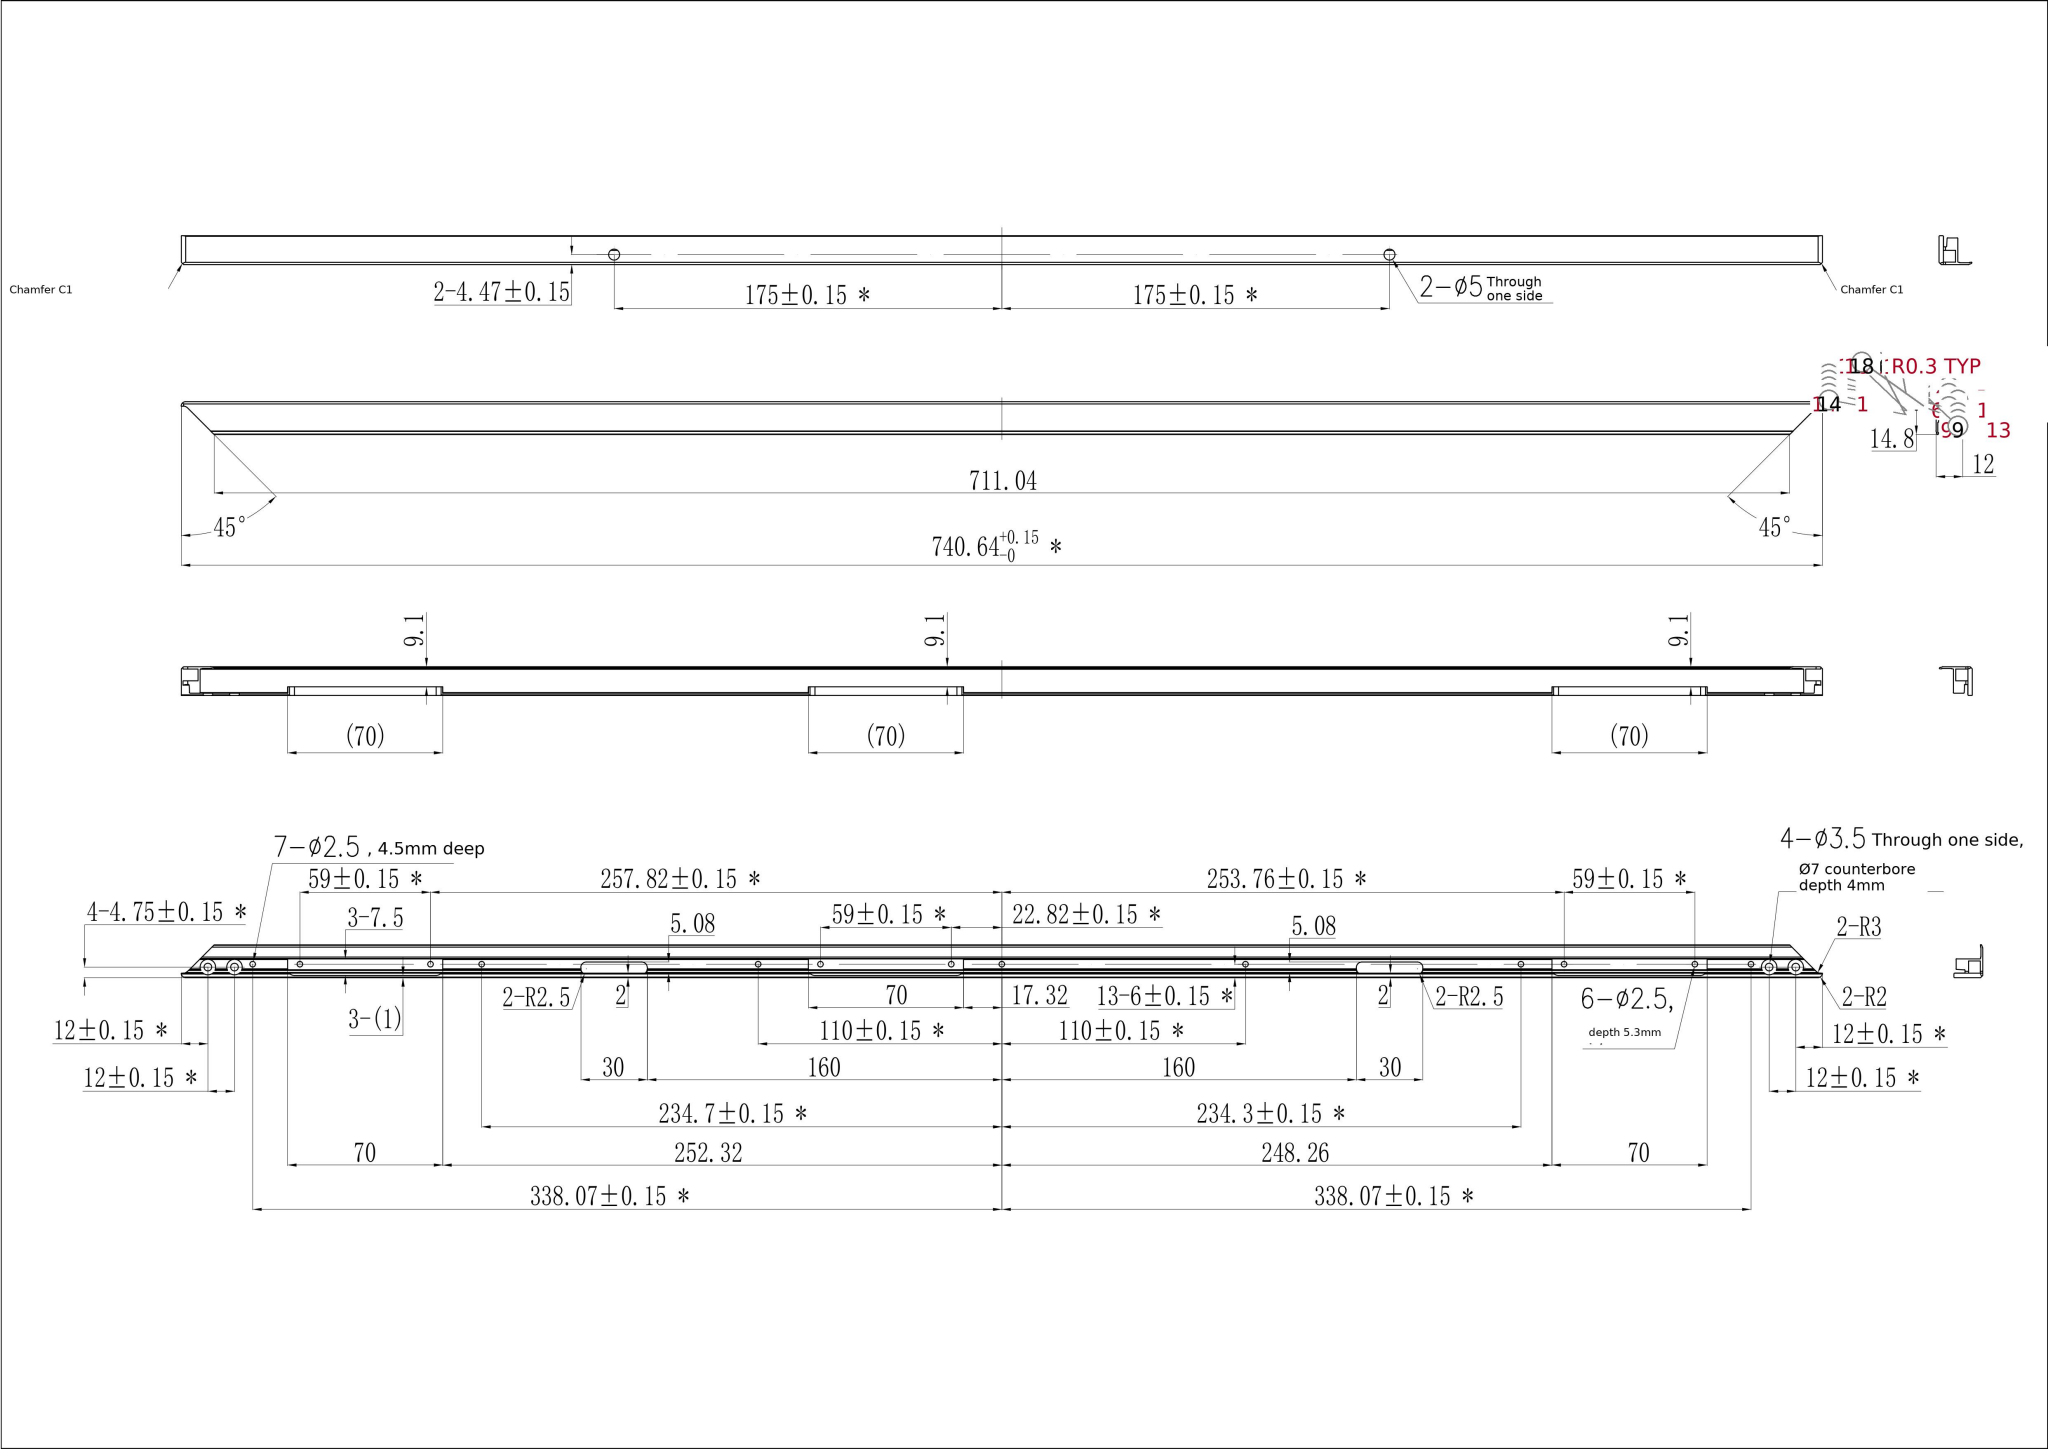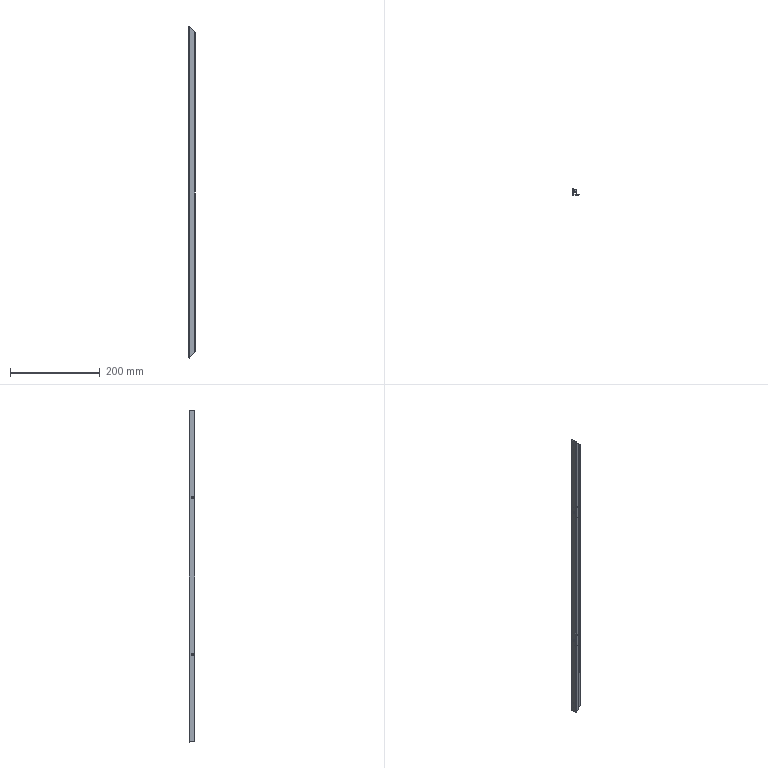Part | SolidWorks | mm | 1 solid | 214 faces | box 14.8 x 13 x 740.64 mm | volume 47193 mm3 | cylinder 125 | plane 89 | commonest cylinder face diameters 0.6 x39 2.5 x26 5 x16 7 x16 6 x16 3.5 x8 4 x2 0.4 x1